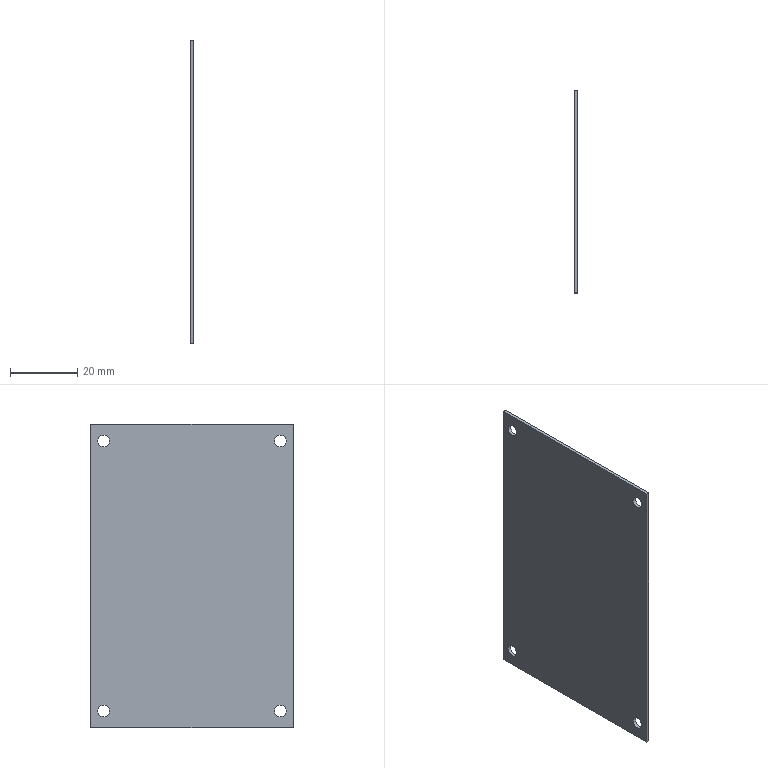Component | NX | COVER_PLATE | 1 solid | 10 faces | box 1 x 60 x 90 mm | volume 5362 mm3 | plane 6 | cylinder 4 | commonest cylinder face diameters 3.5 x4
STEP:
#1=CARTESIAN_POINT('',(0.,0.,0.));
#2=DIRECTION('',(0.,0.,1.));
#3=DIRECTION('',(1.,0.,0.));
#4=AXIS2_PLACEMENT_3D('',#1,#2,#3);
#5=CARTESIAN_POINT('',(-18.838,31.601,36.833));
#6=VERTEX_POINT('',#5);
#7=CARTESIAN_POINT('',(-18.838,-28.399,36.833));
#8=VERTEX_POINT('',#7);
#9=CARTESIAN_POINT('',(-18.838,31.601,36.833));
#10=DIRECTION('',(0.,-1.,0.));
#11=VECTOR('',#10,1.);
#12=LINE('',#9,#11);
#13=CARTESIAN_POINT('',(-19.838,31.601,36.833));
#14=DIRECTION('',(0.,0.,1.));
#15=DIRECTION('',(1.,0.,0.));
#16=AXIS2_PLACEMENT_3D('',#13,#14,#15);
#17=PLANE('',#16);
#18=CARTESIAN_POINT('',(1.,0.));
#19=DIRECTION('',(0.,-1.));
#20=VECTOR('',#19,1.);
#21=LINE('',#18,#20);
#22=(GEOMETRIC_REPRESENTATION_CONTEXT(2)PARAMETRIC_REPRESENTATION_CONTEXT()REPRESENTATION_CONTEXT('',''));
#23=DEFINITIONAL_REPRESENTATION('',(#21),#22);
#24=PCURVE('',#17,#23);
#25=CARTESIAN_POINT('',(-18.838,-24.585,41.833));
#26=DIRECTION('',(-1.,0.,0.));
#27=DIRECTION('',(0.,0.,1.));
#28=AXIS2_PLACEMENT_3D('',#25,#26,#27);
#29=PLANE('',#28);
#30=CARTESIAN_POINT('',(-5.,56.186));
#31=DIRECTION('',(0.,-1.));
#32=VECTOR('',#31,1.);
#33=LINE('',#30,#32);
#34=(GEOMETRIC_REPRESENTATION_CONTEXT(2)PARAMETRIC_REPRESENTATION_CONTEXT()REPRESENTATION_CONTEXT('',''));
#35=DEFINITIONAL_REPRESENTATION('',(#33),#34);
#36=PCURVE('',#29,#35);
#37=SURFACE_CURVE('',#12,(#24,#36),.PCURVE_S1.);
#38=EDGE_CURVE('',#6,#8,#37,.T.);
#39=ORIENTED_EDGE('',*,*,#38,.T.);
#40=CARTESIAN_POINT('',(-19.838,-28.399,36.833));
#41=VERTEX_POINT('',#40);
#42=CARTESIAN_POINT('',(-19.838,-28.399,36.833));
#43=DIRECTION('',(1.,0.,0.));
#44=VECTOR('',#43,1.);
#45=LINE('',#42,#44);
#46=CARTESIAN_POINT('',(0.,-60.));
#47=DIRECTION('',(1.,0.));
#48=VECTOR('',#47,1.);
#49=LINE('',#46,#48);
#50=(GEOMETRIC_REPRESENTATION_CONTEXT(2)PARAMETRIC_REPRESENTATION_CONTEXT()REPRESENTATION_CONTEXT('',''));
#51=DEFINITIONAL_REPRESENTATION('',(#49),#50);
#52=PCURVE('',#17,#51);
#53=CARTESIAN_POINT('',(-19.838,-28.399,36.833));
#54=DIRECTION('',(0.,1.,0.));
#55=DIRECTION('',(-1.,0.,0.));
#56=AXIS2_PLACEMENT_3D('',#53,#54,#55);
#57=PLANE('',#56);
#58=CARTESIAN_POINT('',(0.,0.));
#59=DIRECTION('',(-1.,0.));
#60=VECTOR('',#59,1.);
#61=LINE('',#58,#60);
#62=(GEOMETRIC_REPRESENTATION_CONTEXT(2)PARAMETRIC_REPRESENTATION_CONTEXT()REPRESENTATION_CONTEXT('',''));
#63=DEFINITIONAL_REPRESENTATION('',(#61),#62);
#64=PCURVE('',#57,#63);
#65=SURFACE_CURVE('',#45,(#52,#64),.PCURVE_S1.);
#66=EDGE_CURVE('',#41,#8,#65,.T.);
#67=ORIENTED_EDGE('',*,*,#66,.F.);
#68=CARTESIAN_POINT('',(-19.838,31.601,36.833));
#69=VERTEX_POINT('',#68);
#70=CARTESIAN_POINT('',(-19.838,31.601,36.833));
#71=DIRECTION('',(0.,-1.,0.));
#72=VECTOR('',#71,1.);
#73=LINE('',#70,#72);
#74=CARTESIAN_POINT('',(0.,0.));
#75=DIRECTION('',(0.,-1.));
#76=VECTOR('',#75,1.);
#77=LINE('',#74,#76);
#78=(GEOMETRIC_REPRESENTATION_CONTEXT(2)PARAMETRIC_REPRESENTATION_CONTEXT()REPRESENTATION_CONTEXT('',''));
#79=DEFINITIONAL_REPRESENTATION('',(#77),#78);
#80=PCURVE('',#17,#79);
#81=CARTESIAN_POINT('',(-19.838,-24.585,41.833));
#82=DIRECTION('',(-1.,0.,0.));
#83=DIRECTION('',(0.,0.,1.));
#84=AXIS2_PLACEMENT_3D('',#81,#82,#83);
#85=PLANE('',#84);
#86=CARTESIAN_POINT('',(-5.,56.186));
#87=DIRECTION('',(0.,-1.));
#88=VECTOR('',#87,1.);
#89=LINE('',#86,#88);
#90=(GEOMETRIC_REPRESENTATION_CONTEXT(2)PARAMETRIC_REPRESENTATION_CONTEXT()REPRESENTATION_CONTEXT('',''));
#91=DEFINITIONAL_REPRESENTATION('',(#89),#90);
#92=PCURVE('',#85,#91);
#93=SURFACE_CURVE('',#73,(#80,#92),.PCURVE_S1.);
#94=EDGE_CURVE('',#69,#41,#93,.T.);
#95=ORIENTED_EDGE('',*,*,#94,.F.);
#96=CARTESIAN_POINT('',(-19.838,31.601,36.833));
#97=DIRECTION('',(1.,0.,0.));
#98=VECTOR('',#97,1.);
#99=LINE('',#96,#98);
#100=CARTESIAN_POINT('',(0.,0.));
#101=DIRECTION('',(1.,0.));
#102=VECTOR('',#101,1.);
#103=LINE('',#100,#102);
#104=(GEOMETRIC_REPRESENTATION_CONTEXT(2)PARAMETRIC_REPRESENTATION_CONTEXT()REPRESENTATION_CONTEXT('',''));
#105=DEFINITIONAL_REPRESENTATION('',(#103),#104);
#106=PCURVE('',#17,#105);
#107=CARTESIAN_POINT('',(-19.838,31.601,126.833));
#108=DIRECTION('',(0.,-1.,0.));
#109=DIRECTION('',(1.,0.,0.));
#110=AXIS2_PLACEMENT_3D('',#107,#108,#109);
#111=PLANE('',#110);
#112=CARTESIAN_POINT('',(0.,-90.));
#113=DIRECTION('',(1.,0.));
#114=VECTOR('',#113,1.);
#115=LINE('',#112,#114);
#116=(GEOMETRIC_REPRESENTATION_CONTEXT(2)PARAMETRIC_REPRESENTATION_CONTEXT()REPRESENTATION_CONTEXT('',''));
#117=DEFINITIONAL_REPRESENTATION('',(#115),#116);
#118=PCURVE('',#111,#117);
#119=SURFACE_CURVE('',#99,(#106,#118),.PCURVE_S1.);
#120=EDGE_CURVE('',#69,#6,#119,.T.);
#121=ORIENTED_EDGE('',*,*,#120,.T.);
#122=EDGE_LOOP('',(#39,#67,#95,#121));
#123=FACE_BOUND('',#122,.T.);
#124=ADVANCED_FACE('',(#123),#17,.F.);
#125=CARTESIAN_POINT('',(-18.838,-28.399,126.833));
#126=VERTEX_POINT('',#125);
#127=CARTESIAN_POINT('',(-18.838,-28.399,36.833));
#128=DIRECTION('',(0.,0.,1.));
#129=VECTOR('',#128,1.);
#130=LINE('',#127,#129);
#131=CARTESIAN_POINT('',(-1.,0.));
#132=DIRECTION('',(0.,1.));
#133=VECTOR('',#132,1.);
#134=LINE('',#131,#133);
#135=(GEOMETRIC_REPRESENTATION_CONTEXT(2)PARAMETRIC_REPRESENTATION_CONTEXT()REPRESENTATION_CONTEXT('',''));
#136=DEFINITIONAL_REPRESENTATION('',(#134),#135);
#137=PCURVE('',#57,#136);
#138=CARTESIAN_POINT('',(-5.,-3.814));
#139=DIRECTION('',(1.,0.));
#140=VECTOR('',#139,1.);
#141=LINE('',#138,#140);
#142=(GEOMETRIC_REPRESENTATION_CONTEXT(2)PARAMETRIC_REPRESENTATION_CONTEXT()REPRESENTATION_CONTEXT('',''));
#143=DEFINITIONAL_REPRESENTATION('',(#141),#142);
#144=PCURVE('',#29,#143);
#145=SURFACE_CURVE('',#130,(#137,#144),.PCURVE_S1.);
#146=EDGE_CURVE('',#8,#126,#145,.T.);
#147=ORIENTED_EDGE('',*,*,#146,.T.);
#148=CARTESIAN_POINT('',(-19.838,-28.399,126.833));
#149=VERTEX_POINT('',#148);
#150=CARTESIAN_POINT('',(-19.838,-28.399,126.833));
#151=DIRECTION('',(1.,0.,0.));
#152=VECTOR('',#151,1.);
#153=LINE('',#150,#152);
#154=CARTESIAN_POINT('',(0.,90.));
#155=DIRECTION('',(-1.,0.));
#156=VECTOR('',#155,1.);
#157=LINE('',#154,#156);
#158=(GEOMETRIC_REPRESENTATION_CONTEXT(2)PARAMETRIC_REPRESENTATION_CONTEXT()REPRESENTATION_CONTEXT('',''));
#159=DEFINITIONAL_REPRESENTATION('',(#157),#158);
#160=PCURVE('',#57,#159);
#161=CARTESIAN_POINT('',(-19.838,-28.399,126.833));
#162=DIRECTION('',(0.,0.,-1.));
#163=DIRECTION('',(-1.,0.,0.));
#164=AXIS2_PLACEMENT_3D('',#161,#162,#163);
#165=PLANE('',#164);
#166=CARTESIAN_POINT('',(0.,0.));
#167=DIRECTION('',(-1.,0.));
#168=VECTOR('',#167,1.);
#169=LINE('',#166,#168);
#170=(GEOMETRIC_REPRESENTATION_CONTEXT(2)PARAMETRIC_REPRESENTATION_CONTEXT()REPRESENTATION_CONTEXT('',''));
#171=DEFINITIONAL_REPRESENTATION('',(#169),#170);
#172=PCURVE('',#165,#171);
#173=SURFACE_CURVE('',#153,(#160,#172),.PCURVE_S1.);
#174=EDGE_CURVE('',#149,#126,#173,.T.);
#175=ORIENTED_EDGE('',*,*,#174,.F.);
#176=CARTESIAN_POINT('',(-19.838,-28.399,36.833));
#177=DIRECTION('',(0.,0.,1.));
#178=VECTOR('',#177,1.);
#179=LINE('',#176,#178);
#180=CARTESIAN_POINT('',(0.,0.));
#181=DIRECTION('',(0.,1.));
#182=VECTOR('',#181,1.);
#183=LINE('',#180,#182);
#184=(GEOMETRIC_REPRESENTATION_CONTEXT(2)PARAMETRIC_REPRESENTATION_CONTEXT()REPRESENTATION_CONTEXT('',''));
#185=DEFINITIONAL_REPRESENTATION('',(#183),#184);
#186=PCURVE('',#57,#185);
#187=CARTESIAN_POINT('',(-5.,-3.814));
#188=DIRECTION('',(1.,0.));
#189=VECTOR('',#188,1.);
#190=LINE('',#187,#189);
#191=(GEOMETRIC_REPRESENTATION_CONTEXT(2)PARAMETRIC_REPRESENTATION_CONTEXT()REPRESENTATION_CONTEXT('',''));
#192=DEFINITIONAL_REPRESENTATION('',(#190),#191);
#193=PCURVE('',#85,#192);
#194=SURFACE_CURVE('',#179,(#186,#193),.PCURVE_S1.);
#195=EDGE_CURVE('',#41,#149,#194,.T.);
#196=ORIENTED_EDGE('',*,*,#195,.F.);
#197=ORIENTED_EDGE('',*,*,#66,.T.);
#198=EDGE_LOOP('',(#147,#175,#196,#197));
#199=FACE_BOUND('',#198,.T.);
#200=ADVANCED_FACE('',(#199),#57,.F.);
#201=CARTESIAN_POINT('',(-18.838,31.601,126.833));
#202=VERTEX_POINT('',#201);
#203=CARTESIAN_POINT('',(-18.838,-28.399,126.833));
#204=DIRECTION('',(0.,1.,0.));
#205=VECTOR('',#204,1.);
#206=LINE('',#203,#205);
#207=CARTESIAN_POINT('',(-1.,0.));
#208=DIRECTION('',(0.,1.));
#209=VECTOR('',#208,1.);
#210=LINE('',#207,#209);
#211=(GEOMETRIC_REPRESENTATION_CONTEXT(2)PARAMETRIC_REPRESENTATION_CONTEXT()REPRESENTATION_CONTEXT('',''));
#212=DEFINITIONAL_REPRESENTATION('',(#210),#211);
#213=PCURVE('',#165,#212);
#214=CARTESIAN_POINT('',(85.,-3.814));
#215=DIRECTION('',(0.,1.));
#216=VECTOR('',#215,1.);
#217=LINE('',#214,#216);
#218=(GEOMETRIC_REPRESENTATION_CONTEXT(2)PARAMETRIC_REPRESENTATION_CONTEXT()REPRESENTATION_CONTEXT('',''));
#219=DEFINITIONAL_REPRESENTATION('',(#217),#218);
#220=PCURVE('',#29,#219);
#221=SURFACE_CURVE('',#206,(#213,#220),.PCURVE_S1.);
#222=EDGE_CURVE('',#126,#202,#221,.T.);
#223=ORIENTED_EDGE('',*,*,#222,.T.);
#224=CARTESIAN_POINT('',(-19.838,31.601,126.833));
#225=VERTEX_POINT('',#224);
#226=CARTESIAN_POINT('',(-19.838,31.601,126.833));
#227=DIRECTION('',(1.,0.,0.));
#228=VECTOR('',#227,1.);
#229=LINE('',#226,#228);
#230=CARTESIAN_POINT('',(0.,60.));
#231=DIRECTION('',(-1.,0.));
#232=VECTOR('',#231,1.);
#233=LINE('',#230,#232);
#234=(GEOMETRIC_REPRESENTATION_CONTEXT(2)PARAMETRIC_REPRESENTATION_CONTEXT()REPRESENTATION_CONTEXT('',''));
#235=DEFINITIONAL_REPRESENTATION('',(#233),#234);
#236=PCURVE('',#165,#235);
#237=CARTESIAN_POINT('',(0.,0.));
#238=DIRECTION('',(1.,0.));
#239=VECTOR('',#238,1.);
#240=LINE('',#237,#239);
#241=(GEOMETRIC_REPRESENTATION_CONTEXT(2)PARAMETRIC_REPRESENTATION_CONTEXT()REPRESENTATION_CONTEXT('',''));
#242=DEFINITIONAL_REPRESENTATION('',(#240),#241);
#243=PCURVE('',#111,#242);
#244=SURFACE_CURVE('',#229,(#236,#243),.PCURVE_S1.);
#245=EDGE_CURVE('',#225,#202,#244,.T.);
#246=ORIENTED_EDGE('',*,*,#245,.F.);
#247=CARTESIAN_POINT('',(-19.838,-28.399,126.833));
#248=DIRECTION('',(0.,1.,0.));
#249=VECTOR('',#248,1.);
#250=LINE('',#247,#249);
#251=CARTESIAN_POINT('',(0.,0.));
#252=DIRECTION('',(0.,1.));
#253=VECTOR('',#252,1.);
#254=LINE('',#251,#253);
#255=(GEOMETRIC_REPRESENTATION_CONTEXT(2)PARAMETRIC_REPRESENTATION_CONTEXT()REPRESENTATION_CONTEXT('',''));
#256=DEFINITIONAL_REPRESENTATION('',(#254),#255);
#257=PCURVE('',#165,#256);
#258=CARTESIAN_POINT('',(85.,-3.814));
#259=DIRECTION('',(0.,1.));
#260=VECTOR('',#259,1.);
#261=LINE('',#258,#260);
#262=(GEOMETRIC_REPRESENTATION_CONTEXT(2)PARAMETRIC_REPRESENTATION_CONTEXT()REPRESENTATION_CONTEXT('',''));
#263=DEFINITIONAL_REPRESENTATION('',(#261),#262);
#264=PCURVE('',#85,#263);
#265=SURFACE_CURVE('',#250,(#257,#264),.PCURVE_S1.);
#266=EDGE_CURVE('',#149,#225,#265,.T.);
#267=ORIENTED_EDGE('',*,*,#266,.F.);
#268=ORIENTED_EDGE('',*,*,#174,.T.);
#269=EDGE_LOOP('',(#223,#246,#267,#268));
#270=FACE_BOUND('',#269,.T.);
#271=ADVANCED_FACE('',(#270),#165,.F.);
#272=CARTESIAN_POINT('',(-19.838,-24.585,123.583));
#273=VERTEX_POINT('',#272);
#274=CARTESIAN_POINT('',(-19.838,-24.585,121.833));
#275=DIRECTION('',(-1.,0.,0.));
#276=DIRECTION('',(0.,0.,1.));
#277=AXIS2_PLACEMENT_3D('',#274,#275,#276);
#278=CIRCLE('',#277,1.75);
#279=CARTESIAN_POINT('',(-19.838,-24.585,121.833));
#280=DIRECTION('',(1.,0.,0.));
#281=DIRECTION('',(0.,0.,-1.));
#282=AXIS2_PLACEMENT_3D('',#279,#280,#281);
#283=CYLINDRICAL_SURFACE('',#282,1.75);
#284=CARTESIAN_POINT('',(9.425,0.));
#285=DIRECTION('',(-1.,0.));
#286=VECTOR('',#285,1.);
#287=LINE('',#284,#286);
#288=(GEOMETRIC_REPRESENTATION_CONTEXT(2)PARAMETRIC_REPRESENTATION_CONTEXT()REPRESENTATION_CONTEXT('',''));
#289=DEFINITIONAL_REPRESENTATION('',(#287),#288);
#290=PCURVE('',#283,#289);
#291=CARTESIAN_POINT('',(80.,0.));
#292=DIRECTION('',(1.,0.));
#293=AXIS2_PLACEMENT_2D('',#291,#292);
#294=CIRCLE('',#293,1.75);
#295=(GEOMETRIC_REPRESENTATION_CONTEXT(2)PARAMETRIC_REPRESENTATION_CONTEXT()REPRESENTATION_CONTEXT('',''));
#296=DEFINITIONAL_REPRESENTATION('',(#294),#295);
#297=PCURVE('',#85,#296);
#298=SURFACE_CURVE('',#278,(#290,#297),.PCURVE_S1.);
#299=EDGE_CURVE('',#273,#273,#298,.T.);
#300=ORIENTED_EDGE('',*,*,#299,.F.);
#301=CARTESIAN_POINT('',(-18.838,-24.585,123.583));
#302=VERTEX_POINT('',#301);
#303=CARTESIAN_POINT('',(-19.838,-24.585,123.583));
#304=CARTESIAN_POINT('',(-18.838,-24.585,123.583));
#305=B_SPLINE_CURVE_WITH_KNOTS('',1,(#303,#304),.UNSPECIFIED.,.F.,.F.,(2,2),(0.,1.),.PIECEWISE_BEZIER_KNOTS.);
#306=CARTESIAN_POINT('',(9.425,0.));
#307=DIRECTION('',(0.,1.));
#308=VECTOR('',#307,1.);
#309=LINE('',#306,#308);
#310=(GEOMETRIC_REPRESENTATION_CONTEXT(2)PARAMETRIC_REPRESENTATION_CONTEXT()REPRESENTATION_CONTEXT('',''));
#311=DEFINITIONAL_REPRESENTATION('',(#309),#310);
#312=PCURVE('',#283,#311);
#313=CARTESIAN_POINT('',(3.142,0.));
#314=DIRECTION('',(0.,1.));
#315=VECTOR('',#314,1.);
#316=LINE('',#313,#315);
#317=(GEOMETRIC_REPRESENTATION_CONTEXT(2)PARAMETRIC_REPRESENTATION_CONTEXT()REPRESENTATION_CONTEXT('',''));
#318=DEFINITIONAL_REPRESENTATION('',(#316),#317);
#319=PCURVE('',#283,#318);
#320=SEAM_CURVE('',#305,(#312,#319),.PCURVE_S1.);
#321=EDGE_CURVE('',#273,#302,#320,.T.);
#322=ORIENTED_EDGE('',*,*,#321,.T.);
#323=CARTESIAN_POINT('',(-18.838,-24.585,121.833));
#324=DIRECTION('',(-1.,0.,0.));
#325=DIRECTION('',(0.,0.,1.));
#326=AXIS2_PLACEMENT_3D('',#323,#324,#325);
#327=CIRCLE('',#326,1.75);
#328=CARTESIAN_POINT('',(9.425,1.));
#329=DIRECTION('',(-1.,0.));
#330=VECTOR('',#329,1.);
#331=LINE('',#328,#330);
#332=(GEOMETRIC_REPRESENTATION_CONTEXT(2)PARAMETRIC_REPRESENTATION_CONTEXT()REPRESENTATION_CONTEXT('',''));
#333=DEFINITIONAL_REPRESENTATION('',(#331),#332);
#334=PCURVE('',#283,#333);
#335=CARTESIAN_POINT('',(80.,0.));
#336=DIRECTION('',(1.,0.));
#337=AXIS2_PLACEMENT_2D('',#335,#336);
#338=CIRCLE('',#337,1.75);
#339=(GEOMETRIC_REPRESENTATION_CONTEXT(2)PARAMETRIC_REPRESENTATION_CONTEXT()REPRESENTATION_CONTEXT('',''));
#340=DEFINITIONAL_REPRESENTATION('',(#338),#339);
#341=PCURVE('',#29,#340);
#342=SURFACE_CURVE('',#327,(#334,#341),.PCURVE_S1.);
#343=EDGE_CURVE('',#302,#302,#342,.T.);
#344=ORIENTED_EDGE('',*,*,#343,.T.);
#345=ORIENTED_EDGE('',*,*,#321,.F.);
#346=EDGE_LOOP('',(#300,#322,#344,#345));
#347=FACE_BOUND('',#346,.F.);
#348=ADVANCED_FACE('',(#347),#283,.F.);
#349=CARTESIAN_POINT('',(-19.838,27.786,43.583));
#350=VERTEX_POINT('',#349);
#351=CARTESIAN_POINT('',(-19.838,27.786,41.833));
#352=DIRECTION('',(-1.,0.,0.));
#353=DIRECTION('',(0.,0.,1.));
#354=AXIS2_PLACEMENT_3D('',#351,#352,#353);
#355=CIRCLE('',#354,1.75);
#356=CARTESIAN_POINT('',(-19.838,27.786,41.833));
#357=DIRECTION('',(1.,0.,0.));
#358=DIRECTION('',(0.,0.,-1.));
#359=AXIS2_PLACEMENT_3D('',#356,#357,#358);
#360=CYLINDRICAL_SURFACE('',#359,1.75);
#361=CARTESIAN_POINT('',(9.425,0.));
#362=DIRECTION('',(-1.,0.));
#363=VECTOR('',#362,1.);
#364=LINE('',#361,#363);
#365=(GEOMETRIC_REPRESENTATION_CONTEXT(2)PARAMETRIC_REPRESENTATION_CONTEXT()REPRESENTATION_CONTEXT('',''));
#366=DEFINITIONAL_REPRESENTATION('',(#364),#365);
#367=PCURVE('',#360,#366);
#368=CARTESIAN_POINT('',(0.,52.372));
#369=DIRECTION('',(1.,0.));
#370=AXIS2_PLACEMENT_2D('',#368,#369);
#371=CIRCLE('',#370,1.75);
#372=(GEOMETRIC_REPRESENTATION_CONTEXT(2)PARAMETRIC_REPRESENTATION_CONTEXT()REPRESENTATION_CONTEXT('',''));
#373=DEFINITIONAL_REPRESENTATION('',(#371),#372);
#374=PCURVE('',#85,#373);
#375=SURFACE_CURVE('',#355,(#367,#374),.PCURVE_S1.);
#376=EDGE_CURVE('',#350,#350,#375,.T.);
#377=ORIENTED_EDGE('',*,*,#376,.F.);
#378=CARTESIAN_POINT('',(-18.838,27.786,43.583));
#379=VERTEX_POINT('',#378);
#380=CARTESIAN_POINT('',(-19.838,27.786,43.583));
#381=CARTESIAN_POINT('',(-18.838,27.786,43.583));
#382=B_SPLINE_CURVE_WITH_KNOTS('',1,(#380,#381),.UNSPECIFIED.,.F.,.F.,(2,2),(0.,1.),.PIECEWISE_BEZIER_KNOTS.);
#383=CARTESIAN_POINT('',(9.425,0.));
#384=DIRECTION('',(0.,1.));
#385=VECTOR('',#384,1.);
#386=LINE('',#383,#385);
#387=(GEOMETRIC_REPRESENTATION_CONTEXT(2)PARAMETRIC_REPRESENTATION_CONTEXT()REPRESENTATION_CONTEXT('',''));
#388=DEFINITIONAL_REPRESENTATION('',(#386),#387);
#389=PCURVE('',#360,#388);
#390=CARTESIAN_POINT('',(3.142,0.));
#391=DIRECTION('',(0.,1.));
#392=VECTOR('',#391,1.);
#393=LINE('',#390,#392);
#394=(GEOMETRIC_REPRESENTATION_CONTEXT(2)PARAMETRIC_REPRESENTATION_CONTEXT()REPRESENTATION_CONTEXT('',''));
#395=DEFINITIONAL_REPRESENTATION('',(#393),#394);
#396=PCURVE('',#360,#395);
#397=SEAM_CURVE('',#382,(#389,#396),.PCURVE_S1.);
#398=EDGE_CURVE('',#350,#379,#397,.T.);
#399=ORIENTED_EDGE('',*,*,#398,.T.);
#400=CARTESIAN_POINT('',(-18.838,27.786,41.833));
#401=DIRECTION('',(-1.,0.,0.));
#402=DIRECTION('',(0.,0.,1.));
#403=AXIS2_PLACEMENT_3D('',#400,#401,#402);
#404=CIRCLE('',#403,1.75);
#405=CARTESIAN_POINT('',(9.425,1.));
#406=DIRECTION('',(-1.,0.));
#407=VECTOR('',#406,1.);
#408=LINE('',#405,#407);
#409=(GEOMETRIC_REPRESENTATION_CONTEXT(2)PARAMETRIC_REPRESENTATION_CONTEXT()REPRESENTATION_CONTEXT('',''));
#410=DEFINITIONAL_REPRESENTATION('',(#408),#409);
#411=PCURVE('',#360,#410);
#412=CARTESIAN_POINT('',(0.,52.372));
#413=DIRECTION('',(1.,0.));
#414=AXIS2_PLACEMENT_2D('',#412,#413);
#415=CIRCLE('',#414,1.75);
#416=(GEOMETRIC_REPRESENTATION_CONTEXT(2)PARAMETRIC_REPRESENTATION_CONTEXT()REPRESENTATION_CONTEXT('',''));
#417=DEFINITIONAL_REPRESENTATION('',(#415),#416);
#418=PCURVE('',#29,#417);
#419=SURFACE_CURVE('',#404,(#411,#418),.PCURVE_S1.);
#420=EDGE_CURVE('',#379,#379,#419,.T.);
#421=ORIENTED_EDGE('',*,*,#420,.T.);
#422=ORIENTED_EDGE('',*,*,#398,.F.);
#423=EDGE_LOOP('',(#377,#399,#421,#422));
#424=FACE_BOUND('',#423,.F.);
#425=ADVANCED_FACE('',(#424),#360,.F.);
#426=CARTESIAN_POINT('',(-19.838,-24.585,43.583));
#427=VERTEX_POINT('',#426);
#428=CARTESIAN_POINT('',(-19.838,-24.585,41.833));
#429=DIRECTION('',(-1.,0.,0.));
#430=DIRECTION('',(0.,0.,1.));
#431=AXIS2_PLACEMENT_3D('',#428,#429,#430);
#432=CIRCLE('',#431,1.75);
#433=CARTESIAN_POINT('',(-19.838,-24.585,41.833));
#434=DIRECTION('',(1.,0.,0.));
#435=DIRECTION('',(0.,0.,-1.));
#436=AXIS2_PLACEMENT_3D('',#433,#434,#435);
#437=CYLINDRICAL_SURFACE('',#436,1.75);
#438=CARTESIAN_POINT('',(9.425,0.));
#439=DIRECTION('',(-1.,0.));
#440=VECTOR('',#439,1.);
#441=LINE('',#438,#440);
#442=(GEOMETRIC_REPRESENTATION_CONTEXT(2)PARAMETRIC_REPRESENTATION_CONTEXT()REPRESENTATION_CONTEXT('',''));
#443=DEFINITIONAL_REPRESENTATION('',(#441),#442);
#444=PCURVE('',#437,#443);
#445=CARTESIAN_POINT('',(0.,0.));
#446=DIRECTION('',(1.,0.));
#447=AXIS2_PLACEMENT_2D('',#445,#446);
#448=CIRCLE('',#447,1.75);
#449=(GEOMETRIC_REPRESENTATION_CONTEXT(2)PARAMETRIC_REPRESENTATION_CONTEXT()REPRESENTATION_CONTEXT('',''));
#450=DEFINITIONAL_REPRESENTATION('',(#448),#449);
#451=PCURVE('',#85,#450);
#452=SURFACE_CURVE('',#432,(#444,#451),.PCURVE_S1.);
#453=EDGE_CURVE('',#427,#427,#452,.T.);
#454=ORIENTED_EDGE('',*,*,#453,.F.);
#455=CARTESIAN_POINT('',(-18.838,-24.585,43.583));
#456=VERTEX_POINT('',#455);
#457=CARTESIAN_POINT('',(-19.838,-24.585,43.583));
#458=CARTESIAN_POINT('',(-18.838,-24.585,43.583));
#459=B_SPLINE_CURVE_WITH_KNOTS('',1,(#457,#458),.UNSPECIFIED.,.F.,.F.,(2,2),(0.,1.),.PIECEWISE_BEZIER_KNOTS.);
#460=CARTESIAN_POINT('',(9.425,0.));
#461=DIRECTION('',(0.,1.));
#462=VECTOR('',#461,1.);
#463=LINE('',#460,#462);
#464=(GEOMETRIC_REPRESENTATION_CONTEXT(2)PARAMETRIC_REPRESENTATION_CONTEXT()REPRESENTATION_CONTEXT('',''));
#465=DEFINITIONAL_REPRESENTATION('',(#463),#464);
#466=PCURVE('',#437,#465);
#467=CARTESIAN_POINT('',(3.142,0.));
#468=DIRECTION('',(0.,1.));
#469=VECTOR('',#468,1.);
#470=LINE('',#467,#469);
#471=(GEOMETRIC_REPRESENTATION_CONTEXT(2)PARAMETRIC_REPRESENTATION_CONTEXT()REPRESENTATION_CONTEXT('',''));
#472=DEFINITIONAL_REPRESENTATION('',(#470),#471);
#473=PCURVE('',#437,#472);
#474=SEAM_CURVE('',#459,(#466,#473),.PCURVE_S1.);
#475=EDGE_CURVE('',#427,#456,#474,.T.);
#476=ORIENTED_EDGE('',*,*,#475,.T.);
#477=CARTESIAN_POINT('',(-18.838,-24.585,41.833));
#478=DIRECTION('',(-1.,0.,0.));
#479=DIRECTION('',(0.,0.,1.));
#480=AXIS2_PLACEMENT_3D('',#477,#478,#479);
#481=CIRCLE('',#480,1.75);
#482=CARTESIAN_POINT('',(9.425,1.));
#483=DIRECTION('',(-1.,0.));
#484=VECTOR('',#483,1.);
#485=LINE('',#482,#484);
#486=(GEOMETRIC_REPRESENTATION_CONTEXT(2)PARAMETRIC_REPRESENTATION_CONTEXT()REPRESENTATION_CONTEXT('',''));
#487=DEFINITIONAL_REPRESENTATION('',(#485),#486);
#488=PCURVE('',#437,#487);
#489=CARTESIAN_POINT('',(0.,0.));
#490=DIRECTION('',(1.,0.));
#491=AXIS2_PLACEMENT_2D('',#489,#490);
#492=CIRCLE('',#491,1.75);
#493=(GEOMETRIC_REPRESENTATION_CONTEXT(2)PARAMETRIC_REPRESENTATION_CONTEXT()REPRESENTATION_CONTEXT('',''));
#494=DEFINITIONAL_REPRESENTATION('',(#492),#493);
#495=PCURVE('',#29,#494);
#496=SURFACE_CURVE('',#481,(#488,#495),.PCURVE_S1.);
#497=EDGE_CURVE('',#456,#456,#496,.T.);
#498=ORIENTED_EDGE('',*,*,#497,.T.);
#499=ORIENTED_EDGE('',*,*,#475,.F.);
#500=EDGE_LOOP('',(#454,#476,#498,#499));
#501=FACE_BOUND('',#500,.F.);
#502=ADVANCED_FACE('',(#501),#437,.F.);
#503=CARTESIAN_POINT('',(-18.838,31.601,126.833));
#504=DIRECTION('',(0.,0.,-1.));
#505=VECTOR('',#504,1.);
#506=LINE('',#503,#505);
#507=CARTESIAN_POINT('',(1.,0.));
#508=DIRECTION('',(0.,-1.));
#509=VECTOR('',#508,1.);
#510=LINE('',#507,#509);
#511=(GEOMETRIC_REPRESENTATION_CONTEXT(2)PARAMETRIC_REPRESENTATION_CONTEXT()REPRESENTATION_CONTEXT('',''));
#512=DEFINITIONAL_REPRESENTATION('',(#510),#511);
#513=PCURVE('',#111,#512);
#514=CARTESIAN_POINT('',(85.,56.186));
#515=DIRECTION('',(-1.,0.));
#516=VECTOR('',#515,1.);
#517=LINE('',#514,#516);
#518=(GEOMETRIC_REPRESENTATION_CONTEXT(2)PARAMETRIC_REPRESENTATION_CONTEXT()REPRESENTATION_CONTEXT('',''));
#519=DEFINITIONAL_REPRESENTATION('',(#517),#518);
#520=PCURVE('',#29,#519);
#521=SURFACE_CURVE('',#506,(#513,#520),.PCURVE_S1.);
#522=EDGE_CURVE('',#202,#6,#521,.T.);
#523=ORIENTED_EDGE('',*,*,#522,.T.);
#524=ORIENTED_EDGE('',*,*,#120,.F.);
#525=CARTESIAN_POINT('',(-19.838,31.601,126.833));
#526=DIRECTION('',(0.,0.,-1.));
#527=VECTOR('',#526,1.);
#528=LINE('',#525,#527);
#529=CARTESIAN_POINT('',(0.,0.));
#530=DIRECTION('',(0.,-1.));
#531=VECTOR('',#530,1.);
#532=LINE('',#529,#531);
#533=(GEOMETRIC_REPRESENTATION_CONTEXT(2)PARAMETRIC_REPRESENTATION_CONTEXT()REPRESENTATION_CONTEXT('',''));
#534=DEFINITIONAL_REPRESENTATION('',(#532),#533);
#535=PCURVE('',#111,#534);
#536=CARTESIAN_POINT('',(85.,56.186));
#537=DIRECTION('',(-1.,0.));
#538=VECTOR('',#537,1.);
#539=LINE('',#536,#538);
#540=(GEOMETRIC_REPRESENTATION_CONTEXT(2)PARAMETRIC_REPRESENTATION_CONTEXT()REPRESENTATION_CONTEXT('',''));
#541=DEFINITIONAL_REPRESENTATION('',(#539),#540);
#542=PCURVE('',#85,#541);
#543=SURFACE_CURVE('',#528,(#535,#542),.PCURVE_S1.);
#544=EDGE_CURVE('',#225,#69,#543,.T.);
#545=ORIENTED_EDGE('',*,*,#544,.F.);
#546=ORIENTED_EDGE('',*,*,#245,.T.);
#547=EDGE_LOOP('',(#523,#524,#545,#546));
#548=FACE_BOUND('',#547,.T.);
#549=ADVANCED_FACE('',(#548),#111,.F.);
#550=CARTESIAN_POINT('',(-19.838,27.786,123.583));
#551=VERTEX_POINT('',#550);
#552=CARTESIAN_POINT('',(-19.838,27.786,121.833));
#553=DIRECTION('',(-1.,0.,0.));
#554=DIRECTION('',(0.,0.,1.));
#555=AXIS2_PLACEMENT_3D('',#552,#553,#554);
#556=CIRCLE('',#555,1.75);
#557=CARTESIAN_POINT('',(-19.838,27.786,121.833));
#558=DIRECTION('',(1.,0.,0.));
#559=DIRECTION('',(0.,0.,-1.));
#560=AXIS2_PLACEMENT_3D('',#557,#558,#559);
#561=CYLINDRICAL_SURFACE('',#560,1.75);
#562=CARTESIAN_POINT('',(9.425,0.));
#563=DIRECTION('',(-1.,0.));
#564=VECTOR('',#563,1.);
#565=LINE('',#562,#564);
#566=(GEOMETRIC_REPRESENTATION_CONTEXT(2)PARAMETRIC_REPRESENTATION_CONTEXT()REPRESENTATION_CONTEXT('',''));
#567=DEFINITIONAL_REPRESENTATION('',(#565),#566);
#568=PCURVE('',#561,#567);
#569=CARTESIAN_POINT('',(80.,52.372));
#570=DIRECTION('',(1.,0.));
#571=AXIS2_PLACEMENT_2D('',#569,#570);
#572=CIRCLE('',#571,1.75);
#573=(GEOMETRIC_REPRESENTATION_CONTEXT(2)PARAMETRIC_REPRESENTATION_CONTEXT()REPRESENTATION_CONTEXT('',''));
#574=DEFINITIONAL_REPRESENTATION('',(#572),#573);
#575=PCURVE('',#85,#574);
#576=SURFACE_CURVE('',#556,(#568,#575),.PCURVE_S1.);
#577=EDGE_CURVE('',#551,#551,#576,.T.);
#578=ORIENTED_EDGE('',*,*,#577,.F.);
#579=CARTESIAN_POINT('',(-18.838,27.786,123.583));
#580=VERTEX_POINT('',#579);
#581=CARTESIAN_POINT('',(-19.838,27.786,123.583));
#582=CARTESIAN_POINT('',(-18.838,27.786,123.583));
#583=B_SPLINE_CURVE_WITH_KNOTS('',1,(#581,#582),.UNSPECIFIED.,.F.,.F.,(2,2),(0.,1.),.PIECEWISE_BEZIER_KNOTS.);
#584=CARTESIAN_POINT('',(9.425,0.));
#585=DIRECTION('',(0.,1.));
#586=VECTOR('',#585,1.);
#587=LINE('',#584,#586);
#588=(GEOMETRIC_REPRESENTATION_CONTEXT(2)PARAMETRIC_REPRESENTATION_CONTEXT()REPRESENTATION_CONTEXT('',''));
#589=DEFINITIONAL_REPRESENTATION('',(#587),#588);
#590=PCURVE('',#561,#589);
#591=CARTESIAN_POINT('',(3.142,0.));
#592=DIRECTION('',(0.,1.));
#593=VECTOR('',#592,1.);
#594=LINE('',#591,#593);
#595=(GEOMETRIC_REPRESENTATION_CONTEXT(2)PARAMETRIC_REPRESENTATION_CONTEXT()REPRESENTATION_CONTEXT('',''));
#596=DEFINITIONAL_REPRESENTATION('',(#594),#595);
#597=PCURVE('',#561,#596);
#598=SEAM_CURVE('',#583,(#590,#597),.PCURVE_S1.);
#599=EDGE_CURVE('',#551,#580,#598,.T.);
#600=ORIENTED_EDGE('',*,*,#599,.T.);
#601=CARTESIAN_POINT('',(-18.838,27.786,121.833));
#602=DIRECTION('',(-1.,0.,0.));
#603=DIRECTION('',(0.,0.,1.));
#604=AXIS2_PLACEMENT_3D('',#601,#602,#603);
#605=CIRCLE('',#604,1.75);
#606=CARTESIAN_POINT('',(9.425,1.));
#607=DIRECTION('',(-1.,0.));
#608=VECTOR('',#607,1.);
#609=LINE('',#606,#608);
#610=(GEOMETRIC_REPRESENTATION_CONTEXT(2)PARAMETRIC_REPRESENTATION_CONTEXT()REPRESENTATION_CONTEXT('',''));
#611=DEFINITIONAL_REPRESENTATION('',(#609),#610);
#612=PCURVE('',#561,#611);
#613=CARTESIAN_POINT('',(80.,52.372));
#614=DIRECTION('',(1.,0.));
#615=AXIS2_PLACEMENT_2D('',#613,#614);
#616=CIRCLE('',#615,1.75);
#617=(GEOMETRIC_REPRESENTATION_CONTEXT(2)PARAMETRIC_REPRESENTATION_CONTEXT()REPRESENTATION_CONTEXT('',''));
#618=DEFINITIONAL_REPRESENTATION('',(#616),#617);
#619=PCURVE('',#29,#618);
#620=SURFACE_CURVE('',#605,(#612,#619),.PCURVE_S1.);
#621=EDGE_CURVE('',#580,#580,#620,.T.);
#622=ORIENTED_EDGE('',*,*,#621,.T.);
#623=ORIENTED_EDGE('',*,*,#599,.F.);
#624=EDGE_LOOP('',(#578,#600,#622,#623));
#625=FACE_BOUND('',#624,.F.);
#626=ADVANCED_FACE('',(#625),#561,.F.);
#627=ORIENTED_EDGE('',*,*,#94,.T.);
#628=ORIENTED_EDGE('',*,*,#195,.T.);
#629=ORIENTED_EDGE('',*,*,#266,.T.);
#630=ORIENTED_EDGE('',*,*,#544,.T.);
#631=EDGE_LOOP('',(#627,#628,#629,#630));
#632=FACE_BOUND('',#631,.T.);
#633=ORIENTED_EDGE('',*,*,#453,.F.);
#634=EDGE_LOOP('',(#633));
#635=FACE_BOUND('',#634,.T.);
#636=ORIENTED_EDGE('',*,*,#376,.F.);
#637=EDGE_LOOP('',(#636));
#638=FACE_BOUND('',#637,.T.);
#639=ORIENTED_EDGE('',*,*,#299,.F.);
#640=EDGE_LOOP('',(#639));
#641=FACE_BOUND('',#640,.T.);
#642=ORIENTED_EDGE('',*,*,#577,.F.);
#643=EDGE_LOOP('',(#642));
#644=FACE_BOUND('',#643,.T.);
#645=ADVANCED_FACE('',(#632,#635,#638,#641,#644),#85,.T.);
#646=ORIENTED_EDGE('',*,*,#38,.F.);
#647=ORIENTED_EDGE('',*,*,#522,.F.);
#648=ORIENTED_EDGE('',*,*,#222,.F.);
#649=ORIENTED_EDGE('',*,*,#146,.F.);
#650=EDGE_LOOP('',(#646,#647,#648,#649));
#651=FACE_BOUND('',#650,.T.);
#652=ORIENTED_EDGE('',*,*,#497,.T.);
#653=EDGE_LOOP('',(#652));
#654=FACE_BOUND('',#653,.T.);
#655=ORIENTED_EDGE('',*,*,#420,.T.);
#656=EDGE_LOOP('',(#655));
#657=FACE_BOUND('',#656,.T.);
#658=ORIENTED_EDGE('',*,*,#343,.T.);
#659=EDGE_LOOP('',(#658));
#660=FACE_BOUND('',#659,.T.);
#661=ORIENTED_EDGE('',*,*,#621,.T.);
#662=EDGE_LOOP('',(#661));
#663=FACE_BOUND('',#662,.T.);
#664=ADVANCED_FACE('',(#651,#654,#657,#660,#663),#29,.F.);
#665=CLOSED_SHELL('',(#124,#200,#271,#348,#425,#502,#549,#626,#645,#664));
#666=MANIFOLD_SOLID_BREP('',#665);
#667=(LENGTH_UNIT()NAMED_UNIT(*)SI_UNIT(.MILLI.,.METRE.));
#668=UNCERTAINTY_MEASURE_WITH_UNIT(LENGTH_MEASURE(0.000005),#667,'','');
#669=(NAMED_UNIT(*)PLANE_ANGLE_UNIT()SI_UNIT($,.RADIAN.));
#670=(NAMED_UNIT(*)SI_UNIT($,.STERADIAN.)SOLID_ANGLE_UNIT());
#671=(GEOMETRIC_REPRESENTATION_CONTEXT(3)GLOBAL_UNCERTAINTY_ASSIGNED_CONTEXT((#668))GLOBAL_UNIT_ASSIGNED_CONTEXT((#667,#669,#670))REPRESENTATION_CONTEXT('',''));
#672=ADVANCED_BREP_SHAPE_REPRESENTATION('',(#4,#666),#671);